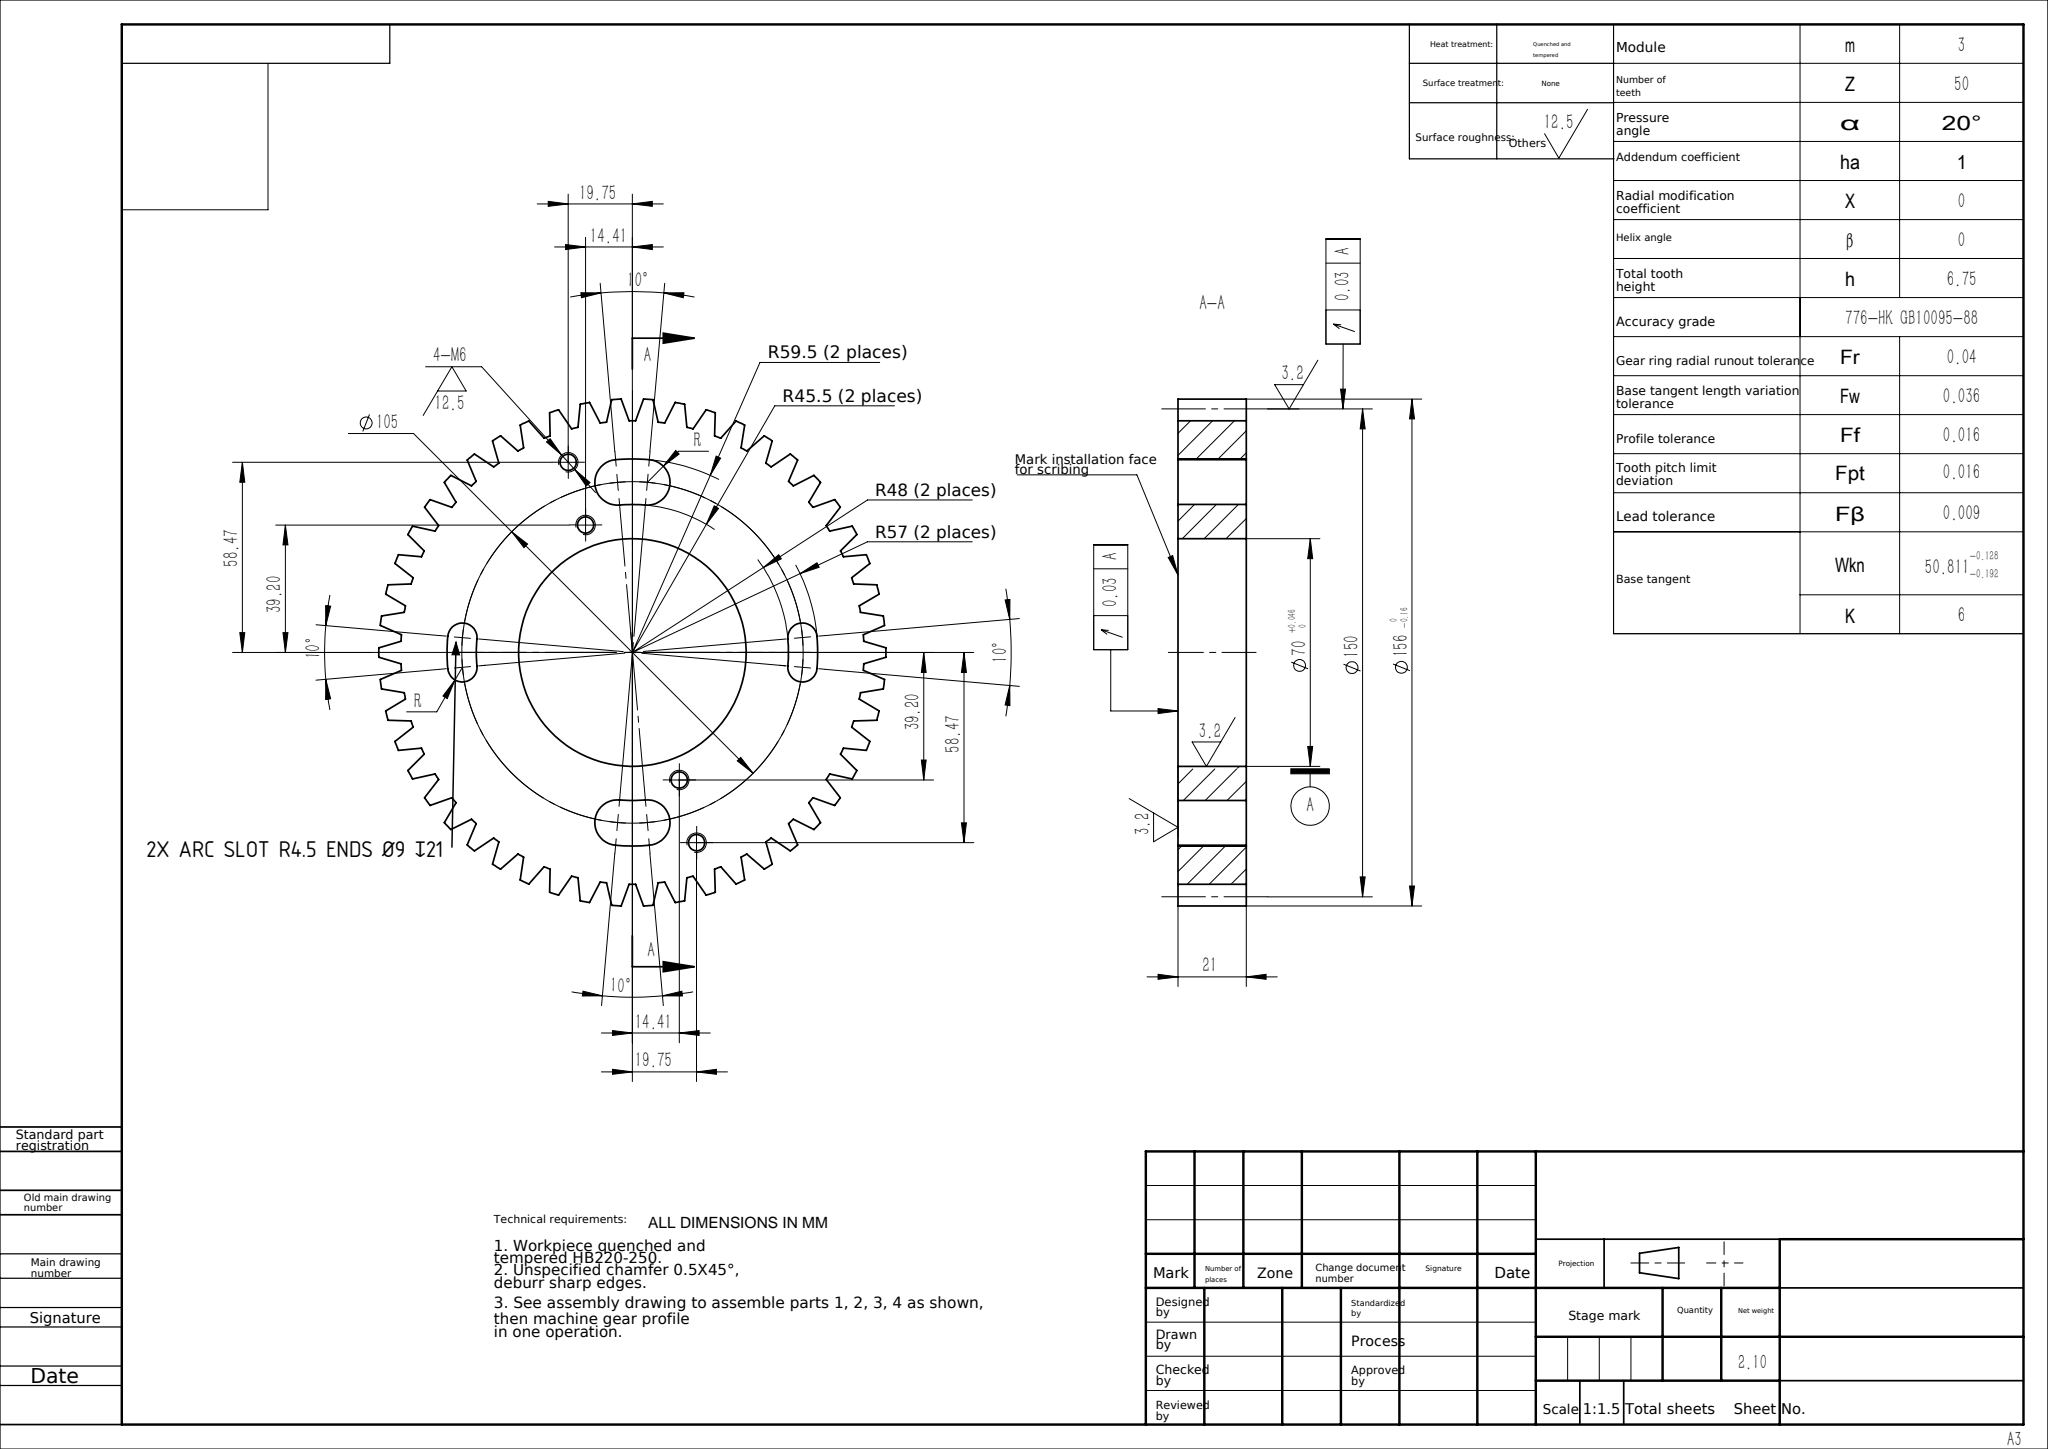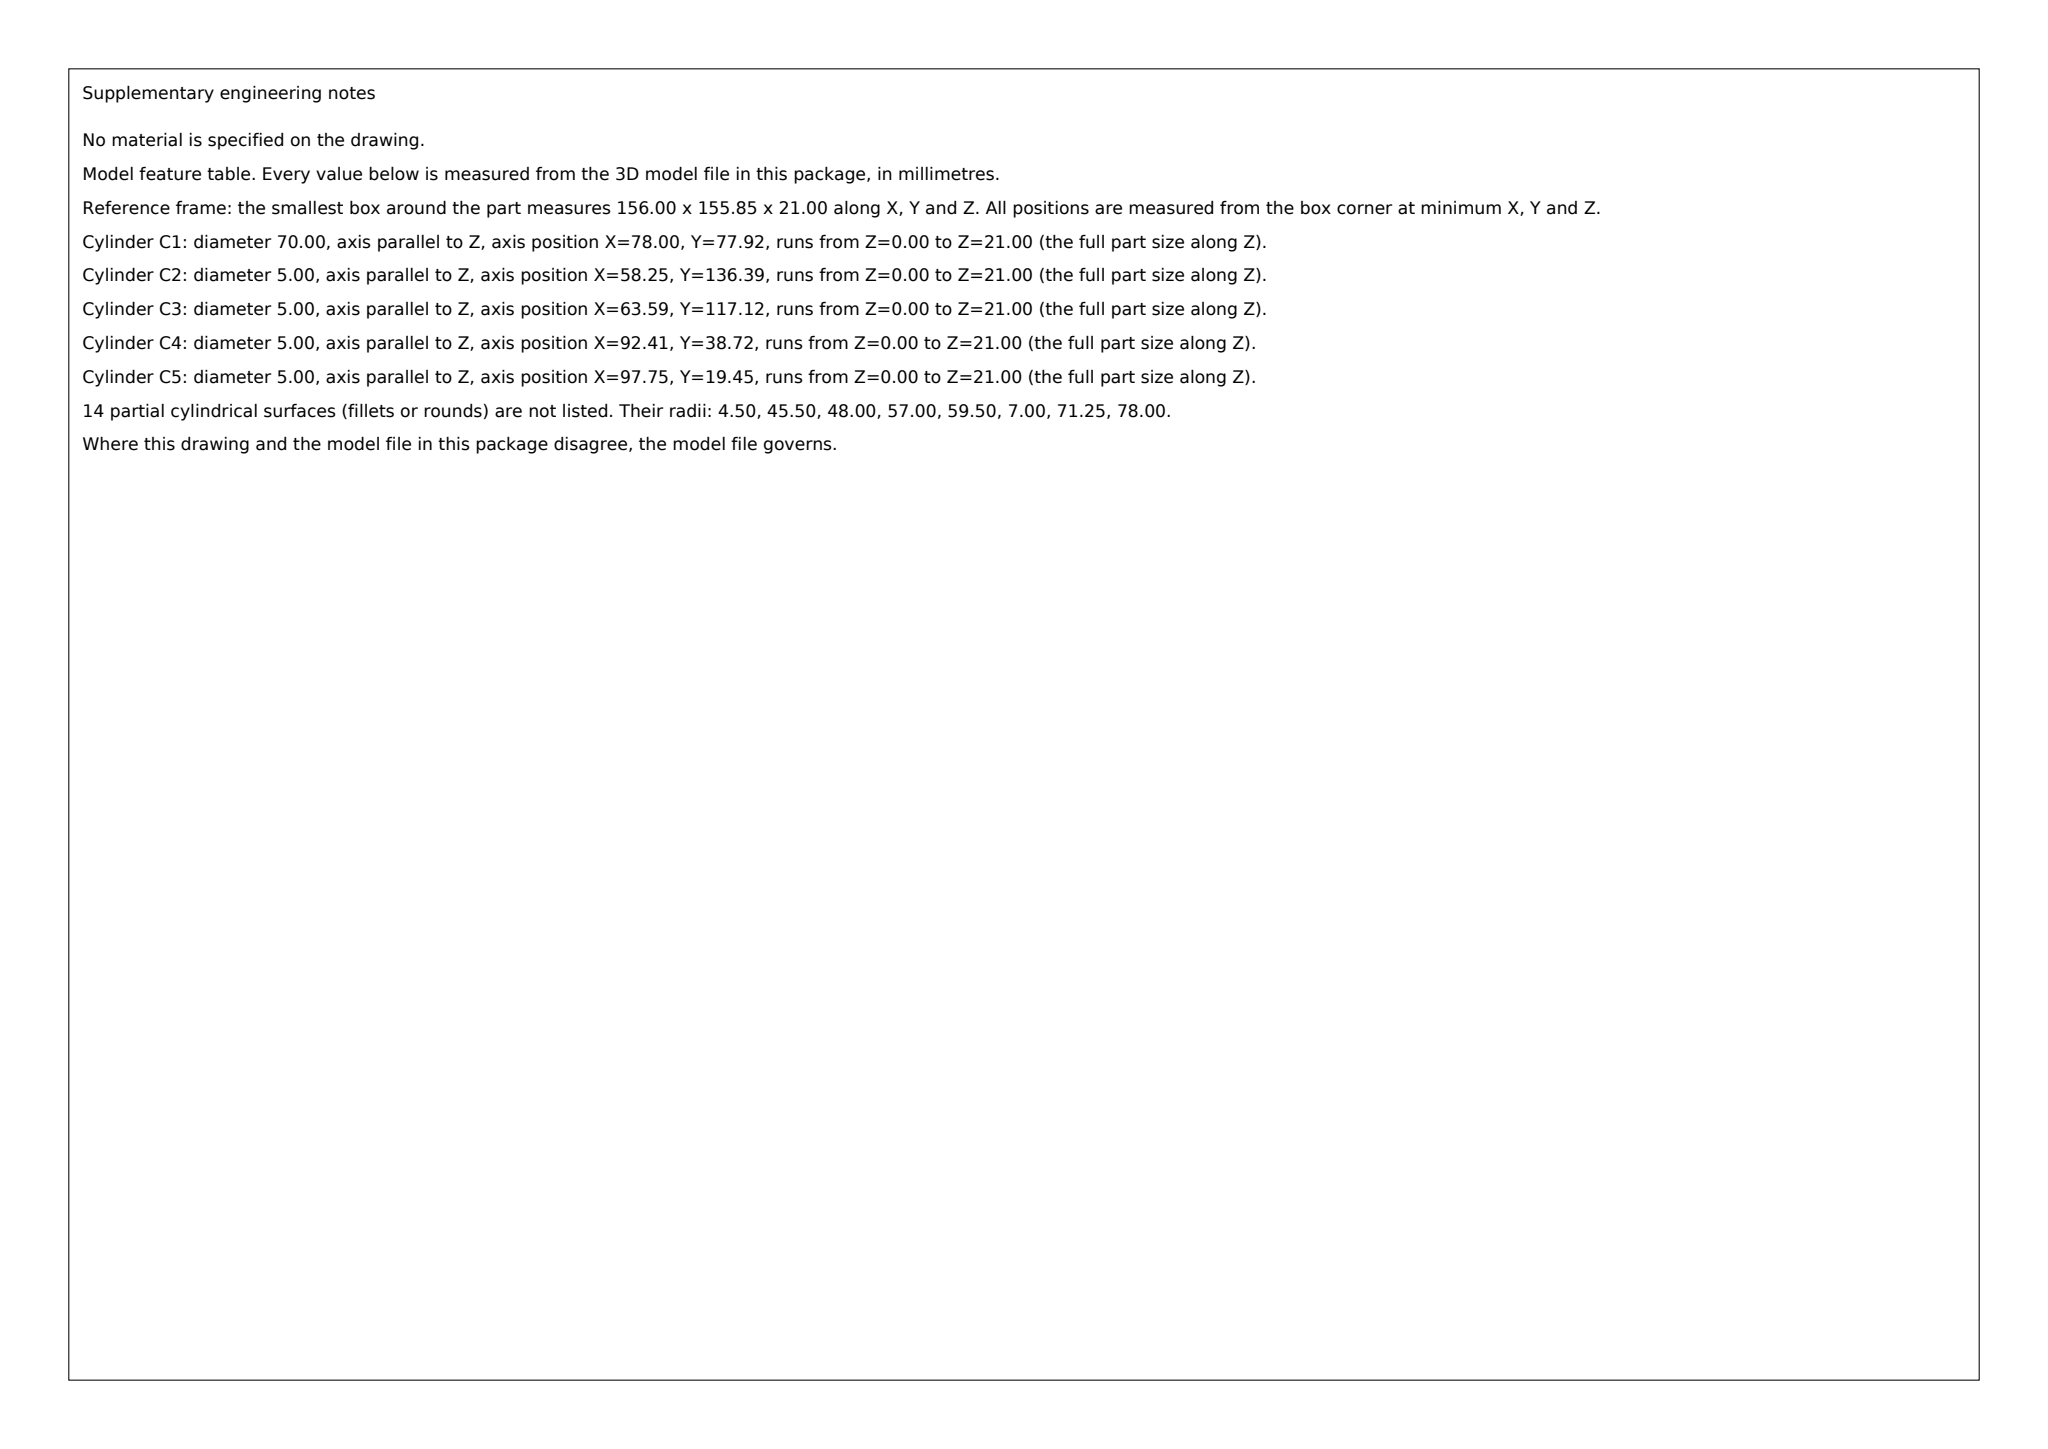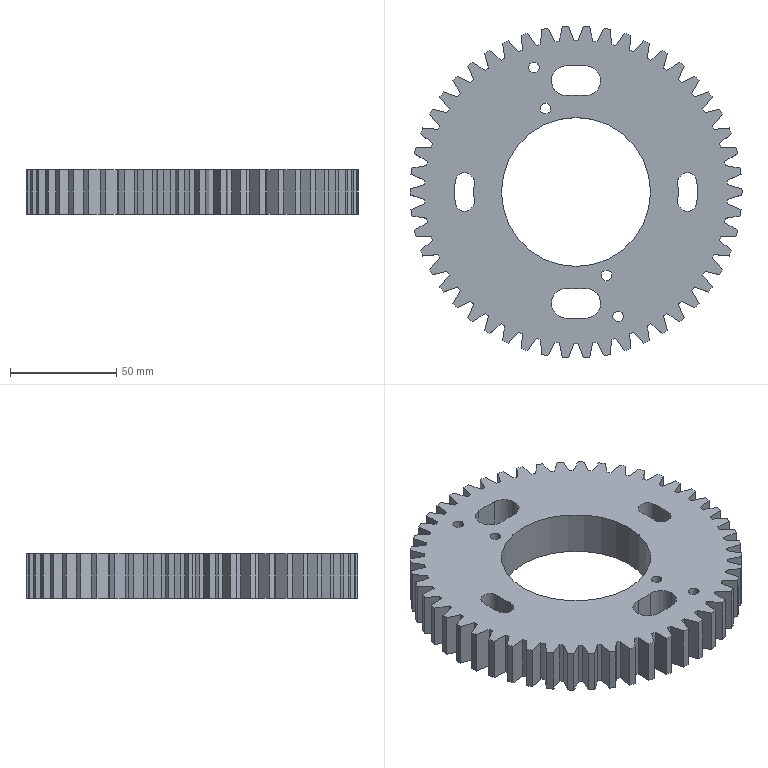Part | SolidWorks | mm | 1 solid | 235 faces | box 156 x 155.85 x 21 mm | volume 269451 mm3 | cylinder 133 | plane 102 | commonest cylinder face diameters 156 x51 142.5 x50 5 x8 9 x8 14 x6 70 x2 91 x2 119 x2
Drawing notes:
2X ARC SLOT, R4.5 ENDS: Ø9 THRU 21 | from the solid: Ø9 z-cylinders at (25.7,73.35),(25.7,82.5),(130.3,73.35),(130.3,82.5), length 21 = full thickness (faces z=0 & z=21)